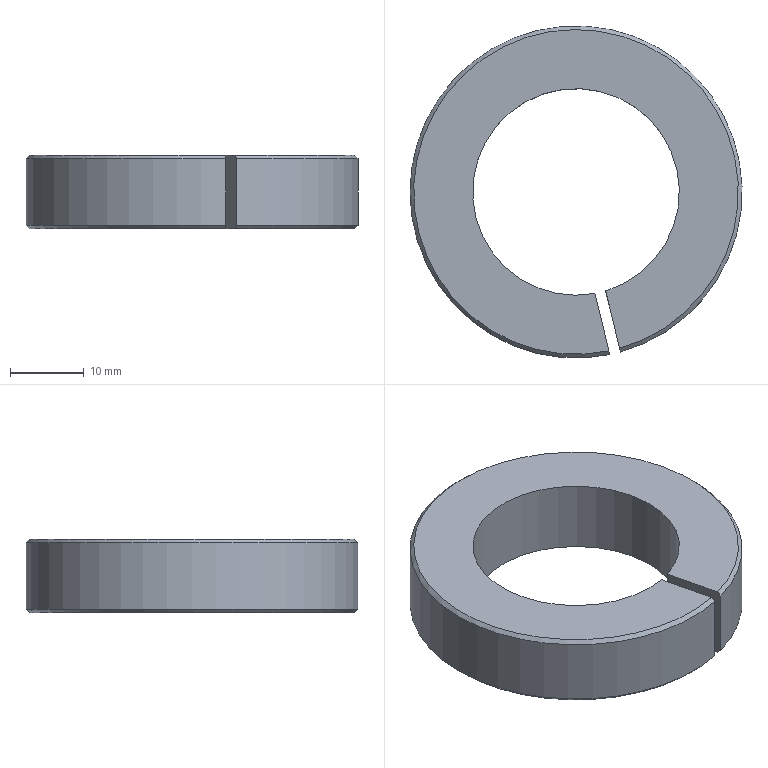Component | SolidWorks | JYTBJ-HeaderRollerBody-1_JYTBJ-LabelLimitSleeve-1 | 1 solid | 9 faces | box 45 x 45 x 10 mm | volume 9585 mm3 | plane 4 | cone 3 | cylinder 2 | commonest cylinder face diameters 45 x1 28 x1
build123d program:
from build123d import *

# Parameters (mm, degrees)
SKETCH1_R           = 22.5
SKETCH1_R_2         = 14
BOSS_EXTRUDE1_DEPTH = 10
SKETCH2_W           = 17.68
SKETCH2_H           = 1.5
CUT_EXTRUDE1_DEPTH  = 34.354
CHAMFER1_SIZE       = 0.5


with BuildPart() as part:
    # Sketch1 → Boss-Extrude1 (new body)
    with BuildSketch(Plane.XY):
        Circle(SKETCH1_R)
        Circle(SKETCH1_R_2, mode=Mode.SUBTRACT)
    extrude(amount=BOSS_EXTRUDE1_DEPTH)

    # Sketch2 → Cut-Extrude1 (cut, through all)
    with BuildSketch(Plane.XY.offset(10)):
        with Locations((-17.235, 0)):
            Rectangle(SKETCH2_W, SKETCH2_H)
    extrude(amount=-CUT_EXTRUDE1_DEPTH, mode=Mode.SUBTRACT)

    # Chamfer1
    chamfer1_edges = [part.edges().sort_by_distance(p)[0] for p in [
        (0.3751, 22.497, 10),
        (0.3751, 22.497, 0),
    ]]
    chamfer(chamfer1_edges, length=CHAMFER1_SIZE)


solid = part.part

# Placed as in the assembly
solid = solid.moved(Location((-199.694, 181.012, 61), (-180, 0, -103.627)))
STEP:
#1=CARTESIAN_POINT('',(-8.066,7.968,2.008));
#2=VERTEX_POINT('',#1);
#3=CARTESIAN_POINT('',(-7.629,6.292,2.008));
#4=VERTEX_POINT('',#3);
#5=CARTESIAN_POINT('',(-7.862,7.126,2.008));
#6=DIRECTION('',(-0.,0.,-1.));
#7=DIRECTION('',(-0.2356,0.9718,0.));
#8=AXIS2_PLACEMENT_3D('',#5,#6,#7);
#9=CIRCLE('',#8,0.8661);
#10=EDGE_CURVE('',#2,#4,#9,.T.);
#11=ORIENTED_EDGE('',*,*,#10,.F.);
#12=CARTESIAN_POINT('',(-8.071,7.987,2.028));
#13=VERTEX_POINT('',#12);
#14=CARTESIAN_POINT('',(-8.071,7.987,2.028));
#15=DIRECTION('',(-0.1666,0.6872,0.7071));
#16=VECTOR('',#15,39.37);
#17=LINE('',#14,#16);
#18=EDGE_CURVE('',#2,#13,#17,.T.);
#19=ORIENTED_EDGE('',*,*,#18,.T.);
#20=CARTESIAN_POINT('',(-7.625,6.273,2.028));
#21=VERTEX_POINT('',#20);
#22=CARTESIAN_POINT('',(-7.862,7.126,2.028));
#23=DIRECTION('',(0.,-0.,1.));
#24=DIRECTION('',(-0.2356,0.9718,0.));
#25=AXIS2_PLACEMENT_3D('',#22,#23,#24);
#26=CIRCLE('',#25,0.8858);
#27=EDGE_CURVE('',#21,#13,#26,.T.);
#28=ORIENTED_EDGE('',*,*,#27,.F.);
#29=CARTESIAN_POINT('',(-7.629,6.292,2.008));
#30=CARTESIAN_POINT('',(-7.628,6.286,2.014));
#31=CARTESIAN_POINT('',(-7.626,6.279,2.021));
#32=CARTESIAN_POINT('',(-7.625,6.273,2.028));
#33=B_SPLINE_CURVE_WITH_KNOTS('',3,(#29,#30,#31,#32),.UNSPECIFIED.,.F.,.F.,(4,4),(0.,0.0007073),.UNSPECIFIED.);
#34=EDGE_CURVE('',#4,#21,#33,.T.);
#35=ORIENTED_EDGE('',*,*,#34,.F.);
#36=EDGE_LOOP('',(#11,#19,#28,#35));
#37=FACE_OUTER_BOUND('',#36,.T.);
#38=CARTESIAN_POINT('',(-7.862,7.126,2.028));
#39=DIRECTION('',(0.,-0.,1.));
#40=DIRECTION('',(-0.2356,0.9718,0.));
#41=AXIS2_PLACEMENT_3D('',#38,#39,#40);
#42=CONICAL_SURFACE('',#41,0.8858,0.7854);
#43=ADVANCED_FACE('',(#37),#42,.T.);
#44=CARTESIAN_POINT('',(-7.629,6.292,2.402));
#45=VERTEX_POINT('',#44);
#46=CARTESIAN_POINT('',(-7.704,6.599,2.402));
#47=VERTEX_POINT('',#46);
#48=CARTESIAN_POINT('',(-7.755,6.812,2.402));
#49=DIRECTION('',(-0.2356,0.9718,0.));
#50=VECTOR('',#49,39.37);
#51=LINE('',#48,#50);
#52=EDGE_CURVE('',#45,#47,#51,.T.);
#53=ORIENTED_EDGE('',*,*,#52,.F.);
#54=CARTESIAN_POINT('',(-7.687,6.278,2.402));
#55=VERTEX_POINT('',#54);
#56=CARTESIAN_POINT('',(-7.862,7.126,2.402));
#57=DIRECTION('',(0.,-0.,1.));
#58=DIRECTION('',(-0.2356,0.9718,0.));
#59=AXIS2_PLACEMENT_3D('',#56,#57,#58);
#60=CIRCLE('',#59,0.8661);
#61=EDGE_CURVE('',#45,#55,#60,.T.);
#62=ORIENTED_EDGE('',*,*,#61,.T.);
#63=CARTESIAN_POINT('',(-7.761,6.585,2.402));
#64=VERTEX_POINT('',#63);
#65=CARTESIAN_POINT('',(-7.649,6.122,2.402));
#66=DIRECTION('',(0.2356,-0.9718,-0.));
#67=VECTOR('',#66,39.37);
#68=LINE('',#65,#67);
#69=EDGE_CURVE('',#64,#55,#68,.T.);
#70=ORIENTED_EDGE('',*,*,#69,.F.);
#71=CARTESIAN_POINT('',(-7.862,7.126,2.402));
#72=DIRECTION('',(0.,-0.,1.));
#73=DIRECTION('',(-0.2356,0.9718,0.));
#74=AXIS2_PLACEMENT_3D('',#71,#72,#73);
#75=CIRCLE('',#74,0.5512);
#76=EDGE_CURVE('',#47,#64,#75,.T.);
#77=ORIENTED_EDGE('',*,*,#76,.F.);
#78=EDGE_LOOP('',(#53,#62,#70,#77));
#79=FACE_OUTER_BOUND('',#78,.T.);
#80=CARTESIAN_POINT('',(-7.862,7.126,2.402));
#81=DIRECTION('',(0.,-0.,1.));
#82=DIRECTION('',(-0.2356,0.9718,0.));
#83=AXIS2_PLACEMENT_3D('',#80,#81,#82);
#84=PLANE('',#83);
#85=ADVANCED_FACE('',(#79),#84,.T.);
#86=CARTESIAN_POINT('',(-7.761,6.585,2.008));
#87=VERTEX_POINT('',#86);
#88=CARTESIAN_POINT('',(-7.687,6.278,2.008));
#89=VERTEX_POINT('',#88);
#90=CARTESIAN_POINT('',(-7.649,6.122,2.008));
#91=DIRECTION('',(0.2356,-0.9718,-0.));
#92=VECTOR('',#91,39.37);
#93=LINE('',#90,#92);
#94=EDGE_CURVE('',#87,#89,#93,.T.);
#95=ORIENTED_EDGE('',*,*,#94,.T.);
#96=CARTESIAN_POINT('',(-7.862,7.126,2.008));
#97=DIRECTION('',(-0.,0.,-1.));
#98=DIRECTION('',(-0.2356,0.9718,0.));
#99=AXIS2_PLACEMENT_3D('',#96,#97,#98);
#100=CIRCLE('',#99,0.8661);
#101=EDGE_CURVE('',#89,#2,#100,.T.);
#102=ORIENTED_EDGE('',*,*,#101,.T.);
#103=ORIENTED_EDGE('',*,*,#10,.T.);
#104=CARTESIAN_POINT('',(-7.704,6.599,2.008));
#105=VERTEX_POINT('',#104);
#106=CARTESIAN_POINT('',(-7.755,6.812,2.008));
#107=DIRECTION('',(-0.2356,0.9718,0.));
#108=VECTOR('',#107,39.37);
#109=LINE('',#106,#108);
#110=EDGE_CURVE('',#4,#105,#109,.T.);
#111=ORIENTED_EDGE('',*,*,#110,.T.);
#112=CARTESIAN_POINT('',(-7.862,7.126,2.008));
#113=DIRECTION('',(0.,-0.,1.));
#114=DIRECTION('',(-0.2356,0.9718,0.));
#115=AXIS2_PLACEMENT_3D('',#112,#113,#114);
#116=CIRCLE('',#115,0.5512);
#117=EDGE_CURVE('',#105,#87,#116,.T.);
#118=ORIENTED_EDGE('',*,*,#117,.T.);
#119=EDGE_LOOP('',(#95,#102,#103,#111,#118));
#120=FACE_OUTER_BOUND('',#119,.T.);
#121=CARTESIAN_POINT('',(-7.862,7.126,2.008));
#122=DIRECTION('',(0.,-0.,1.));
#123=DIRECTION('',(-0.2356,0.9718,0.));
#124=AXIS2_PLACEMENT_3D('',#121,#122,#123);
#125=PLANE('',#124);
#126=ADVANCED_FACE('',(#120),#125,.F.);
#127=CARTESIAN_POINT('',(-7.682,6.259,2.028));
#128=VERTEX_POINT('',#127);
#129=CARTESIAN_POINT('',(-7.682,6.259,2.382));
#130=VERTEX_POINT('',#129);
#131=CARTESIAN_POINT('',(-7.682,6.259,2.402));
#132=DIRECTION('',(0.,-0.,1.));
#133=VECTOR('',#132,39.37);
#134=LINE('',#131,#133);
#135=EDGE_CURVE('',#128,#130,#134,.T.);
#136=ORIENTED_EDGE('',*,*,#135,.T.);
#137=CARTESIAN_POINT('',(-7.625,6.273,2.382));
#138=VERTEX_POINT('',#137);
#139=CARTESIAN_POINT('',(-7.862,7.126,2.382));
#140=DIRECTION('',(-0.,0.,-1.));
#141=DIRECTION('',(-0.2356,0.9718,0.));
#142=AXIS2_PLACEMENT_3D('',#139,#140,#141);
#143=CIRCLE('',#142,0.8858);
#144=EDGE_CURVE('',#130,#138,#143,.T.);
#145=ORIENTED_EDGE('',*,*,#144,.T.);
#146=CARTESIAN_POINT('',(-7.625,6.273,2.402));
#147=DIRECTION('',(-0.,0.,-1.));
#148=VECTOR('',#147,39.37);
#149=LINE('',#146,#148);
#150=EDGE_CURVE('',#138,#21,#149,.T.);
#151=ORIENTED_EDGE('',*,*,#150,.T.);
#152=ORIENTED_EDGE('',*,*,#27,.T.);
#153=CARTESIAN_POINT('',(-7.862,7.126,2.028));
#154=DIRECTION('',(0.,-0.,1.));
#155=DIRECTION('',(-0.2356,0.9718,0.));
#156=AXIS2_PLACEMENT_3D('',#153,#154,#155);
#157=CIRCLE('',#156,0.8858);
#158=EDGE_CURVE('',#13,#128,#157,.T.);
#159=ORIENTED_EDGE('',*,*,#158,.T.);
#160=EDGE_LOOP('',(#136,#145,#151,#152,#159));
#161=FACE_OUTER_BOUND('',#160,.T.);
#162=CARTESIAN_POINT('',(-7.862,7.126,2.402));
#163=DIRECTION('',(-0.,0.,-1.));
#164=DIRECTION('',(0.2356,-0.9718,0.));
#165=AXIS2_PLACEMENT_3D('',#162,#163,#164);
#166=CYLINDRICAL_SURFACE('',#165,0.8858);
#167=ADVANCED_FACE('',(#161),#166,.T.);
#168=CARTESIAN_POINT('',(-7.761,6.585,2.402));
#169=DIRECTION('',(0.,-0.,1.));
#170=VECTOR('',#169,39.37);
#171=LINE('',#168,#170);
#172=EDGE_CURVE('',#87,#64,#171,.T.);
#173=ORIENTED_EDGE('',*,*,#172,.F.);
#174=ORIENTED_EDGE('',*,*,#117,.F.);
#175=CARTESIAN_POINT('',(-7.704,6.599,2.402));
#176=DIRECTION('',(-0.,0.,-1.));
#177=VECTOR('',#176,39.37);
#178=LINE('',#175,#177);
#179=EDGE_CURVE('',#47,#105,#178,.T.);
#180=ORIENTED_EDGE('',*,*,#179,.F.);
#181=ORIENTED_EDGE('',*,*,#76,.T.);
#182=EDGE_LOOP('',(#173,#174,#180,#181));
#183=FACE_OUTER_BOUND('',#182,.T.);
#184=CARTESIAN_POINT('',(-7.862,7.126,2.402));
#185=DIRECTION('',(-0.,0.,-1.));
#186=DIRECTION('',(0.2356,-0.9718,0.));
#187=AXIS2_PLACEMENT_3D('',#184,#185,#186);
#188=CYLINDRICAL_SURFACE('',#187,0.5512);
#189=ADVANCED_FACE('',(#183),#188,.F.);
#190=ORIENTED_EDGE('',*,*,#150,.F.);
#191=CARTESIAN_POINT('',(-7.625,6.273,2.382));
#192=CARTESIAN_POINT('',(-7.626,6.279,2.388));
#193=CARTESIAN_POINT('',(-7.628,6.286,2.395));
#194=CARTESIAN_POINT('',(-7.629,6.292,2.402));
#195=B_SPLINE_CURVE_WITH_KNOTS('',3,(#191,#192,#193,#194),.UNSPECIFIED.,.F.,.F.,(4,4),(0.,0.0007073),.UNSPECIFIED.);
#196=EDGE_CURVE('',#138,#45,#195,.T.);
#197=ORIENTED_EDGE('',*,*,#196,.T.);
#198=ORIENTED_EDGE('',*,*,#52,.T.);
#199=ORIENTED_EDGE('',*,*,#179,.T.);
#200=ORIENTED_EDGE('',*,*,#110,.F.);
#201=ORIENTED_EDGE('',*,*,#34,.T.);
#202=EDGE_LOOP('',(#190,#197,#198,#199,#200,#201));
#203=FACE_OUTER_BOUND('',#202,.T.);
#204=CARTESIAN_POINT('',(-7.755,6.812,2.008));
#205=DIRECTION('',(0.9718,0.2356,0.));
#206=DIRECTION('',(-0.2356,0.9718,0.));
#207=AXIS2_PLACEMENT_3D('',#204,#205,#206);
#208=PLANE('',#207);
#209=ADVANCED_FACE('',(#203),#208,.F.);
#210=ORIENTED_EDGE('',*,*,#69,.T.);
#211=CARTESIAN_POINT('',(-7.687,6.278,2.402));
#212=CARTESIAN_POINT('',(-7.685,6.272,2.395));
#213=CARTESIAN_POINT('',(-7.684,6.265,2.388));
#214=CARTESIAN_POINT('',(-7.682,6.259,2.382));
#215=B_SPLINE_CURVE_WITH_KNOTS('',3,(#211,#212,#213,#214),.UNSPECIFIED.,.F.,.F.,(4,4),(0.,0.0007073),.UNSPECIFIED.);
#216=EDGE_CURVE('',#55,#130,#215,.T.);
#217=ORIENTED_EDGE('',*,*,#216,.T.);
#218=ORIENTED_EDGE('',*,*,#135,.F.);
#219=CARTESIAN_POINT('',(-7.682,6.259,2.028));
#220=CARTESIAN_POINT('',(-7.684,6.265,2.021));
#221=CARTESIAN_POINT('',(-7.685,6.272,2.014));
#222=CARTESIAN_POINT('',(-7.687,6.278,2.008));
#223=B_SPLINE_CURVE_WITH_KNOTS('',3,(#219,#220,#221,#222),.UNSPECIFIED.,.F.,.F.,(4,4),(0.,0.0007073),.UNSPECIFIED.);
#224=EDGE_CURVE('',#128,#89,#223,.T.);
#225=ORIENTED_EDGE('',*,*,#224,.T.);
#226=ORIENTED_EDGE('',*,*,#94,.F.);
#227=ORIENTED_EDGE('',*,*,#172,.T.);
#228=EDGE_LOOP('',(#210,#217,#218,#225,#226,#227));
#229=FACE_OUTER_BOUND('',#228,.T.);
#230=CARTESIAN_POINT('',(-7.649,6.122,2.008));
#231=DIRECTION('',(-0.9718,-0.2356,-0.));
#232=DIRECTION('',(0.,-0.,1.));
#233=AXIS2_PLACEMENT_3D('',#230,#231,#232);
#234=PLANE('',#233);
#235=ADVANCED_FACE('',(#229),#234,.F.);
#236=ORIENTED_EDGE('',*,*,#196,.F.);
#237=ORIENTED_EDGE('',*,*,#144,.F.);
#238=ORIENTED_EDGE('',*,*,#216,.F.);
#239=ORIENTED_EDGE('',*,*,#61,.F.);
#240=EDGE_LOOP('',(#236,#237,#238,#239));
#241=FACE_OUTER_BOUND('',#240,.T.);
#242=CARTESIAN_POINT('',(-7.862,7.126,2.402));
#243=DIRECTION('',(-0.,0.,-1.));
#244=DIRECTION('',(0.2356,-0.9718,0.));
#245=AXIS2_PLACEMENT_3D('',#242,#243,#244);
#246=CONICAL_SURFACE('',#245,0.8661,0.7854);
#247=ADVANCED_FACE('',(#241),#246,.T.);
#248=ORIENTED_EDGE('',*,*,#18,.F.);
#249=ORIENTED_EDGE('',*,*,#101,.F.);
#250=ORIENTED_EDGE('',*,*,#224,.F.);
#251=ORIENTED_EDGE('',*,*,#158,.F.);
#252=EDGE_LOOP('',(#248,#249,#250,#251));
#253=FACE_OUTER_BOUND('',#252,.T.);
#254=CARTESIAN_POINT('',(-7.862,7.126,2.028));
#255=DIRECTION('',(0.,-0.,1.));
#256=DIRECTION('',(-0.2356,0.9718,0.));
#257=AXIS2_PLACEMENT_3D('',#254,#255,#256);
#258=CONICAL_SURFACE('',#257,0.8858,0.7854);
#259=ADVANCED_FACE('',(#253),#258,.T.);
#260=CLOSED_SHELL('',(#43,#85,#126,#167,#189,#209,#235,#247,#259));
#261=MANIFOLD_SOLID_BREP('',#260);
#262=CARTESIAN_POINT('',(0.,0.,0.));
#263=DIRECTION('',(0.,0.,1.));
#264=DIRECTION('',(1.,0.,0.));
#265=AXIS2_PLACEMENT_3D('',#262,#263,#264);
#266=(LENGTH_UNIT()NAMED_UNIT(*)SI_UNIT($,.METRE.));
#267=LENGTH_MEASURE_WITH_UNIT(LENGTH_MEASURE(0.0254),#266);
#268=DIMENSIONAL_EXPONENTS(1.,0.,0.,0.,0.,0.,0.);
#269=(CONVERSION_BASED_UNIT('',#267)LENGTH_UNIT()NAMED_UNIT(#268));
#270=UNCERTAINTY_MEASURE_WITH_UNIT(LENGTH_MEASURE(0.00001),#269,'','');
#271=(NAMED_UNIT(*)PLANE_ANGLE_UNIT()SI_UNIT($,.RADIAN.));
#272=(NAMED_UNIT(*)SI_UNIT($,.STERADIAN.)SOLID_ANGLE_UNIT());
#273=(GEOMETRIC_REPRESENTATION_CONTEXT(3)GLOBAL_UNCERTAINTY_ASSIGNED_CONTEXT((#270))GLOBAL_UNIT_ASSIGNED_CONTEXT((#269,#271,#272))REPRESENTATION_CONTEXT('',''));
#274=ADVANCED_BREP_SHAPE_REPRESENTATION('',(#261,#265),#273);
#275=COLOUR_RGB('',0.7922,0.8196,0.9333);
#276=FILL_AREA_STYLE_COLOUR('',#275);
#277=FILL_AREA_STYLE('',(#276));
#278=SURFACE_STYLE_FILL_AREA(#277);
#279=SURFACE_SIDE_STYLE('',(#278));
#280=SURFACE_STYLE_USAGE(.BOTH.,#279);
#281=PRESENTATION_STYLE_ASSIGNMENT((#280));
#282=STYLED_ITEM('',(#281),#261);
#283=(LENGTH_UNIT()NAMED_UNIT(*)SI_UNIT($,.METRE.));
#284=LENGTH_MEASURE_WITH_UNIT(LENGTH_MEASURE(0.0254),#283);
#285=DIMENSIONAL_EXPONENTS(1.,0.,0.,0.,0.,0.,0.);
#286=(CONVERSION_BASED_UNIT('',#284)LENGTH_UNIT()NAMED_UNIT(#285));
#287=UNCERTAINTY_MEASURE_WITH_UNIT(LENGTH_MEASURE(0.00001),#286,'','');
#288=(NAMED_UNIT(*)PLANE_ANGLE_UNIT()SI_UNIT($,.RADIAN.));
#289=(NAMED_UNIT(*)SI_UNIT($,.STERADIAN.)SOLID_ANGLE_UNIT());
#290=(GEOMETRIC_REPRESENTATION_CONTEXT(3)GLOBAL_UNCERTAINTY_ASSIGNED_CONTEXT((#287))GLOBAL_UNIT_ASSIGNED_CONTEXT((#286,#288,#289))REPRESENTATION_CONTEXT('',''));
#291=MECHANICAL_DESIGN_GEOMETRIC_PRESENTATION_REPRESENTATION('',(#282),#290);
#292=PRESENTATION_LAYER_ASSIGNMENT('','',(#282));